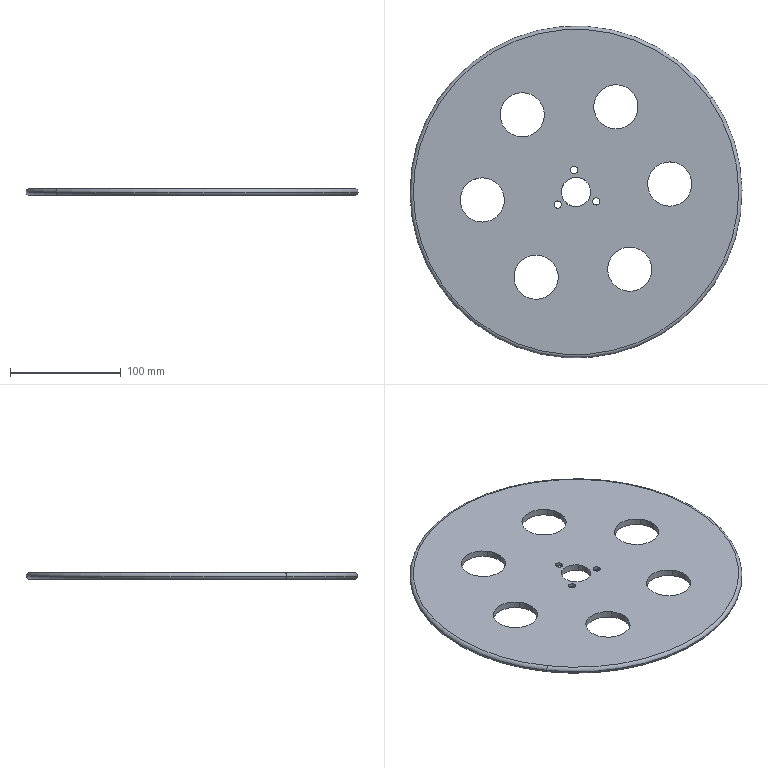Component | SolidWorks | JYTBJ-HeaderPlate-1 | 1 solid | 32 faces | box 300 x 300 x 6 mm | volume 370827 mm3 | cylinder 20 | cone 6 | torus 4 | plane 2 | commonest cylinder face diameters 40 x12 6.6 x6 26.5 x2
STEP:
#1=COLOUR_RGB('',0.7922,0.8196,0.9333);
#2=FILL_AREA_STYLE_COLOUR('',#1);
#3=FILL_AREA_STYLE('',(#2));
#4=SURFACE_STYLE_FILL_AREA(#3);
#5=SURFACE_SIDE_STYLE('',(#4));
#6=SURFACE_STYLE_USAGE(.BOTH.,#5);
#7=PRESENTATION_STYLE_ASSIGNMENT((#6));
#8=CARTESIAN_POINT('',(-2.556,3.98,1.909));
#9=VERTEX_POINT('',#8);
#10=CARTESIAN_POINT('',(-3.848,3.08,1.909));
#11=VERTEX_POINT('',#10);
#12=CARTESIAN_POINT('',(-3.202,3.53,1.909));
#13=DIRECTION('',(0.,0.,-1.));
#14=DIRECTION('',(0.08494,-0.9964,0.));
#15=AXIS2_PLACEMENT_3D('',#12,#13,#14);
#16=CIRCLE('',#15,0.7874);
#17=EDGE_CURVE('',#9,#11,#16,.T.);
#18=ORIENTED_EDGE('',*,*,#17,.F.);
#19=CARTESIAN_POINT('',(-2.556,3.98,1.673));
#20=VERTEX_POINT('',#19);
#21=CARTESIAN_POINT('',(-2.556,3.98,1.909));
#22=DIRECTION('',(0.,0.,-1.));
#23=VECTOR('',#22,39.37);
#24=LINE('',#21,#23);
#25=EDGE_CURVE('',#9,#20,#24,.T.);
#26=ORIENTED_EDGE('',*,*,#25,.T.);
#27=CARTESIAN_POINT('',(-3.848,3.08,1.673));
#28=VERTEX_POINT('',#27);
#29=CARTESIAN_POINT('',(-3.202,3.53,1.673));
#30=DIRECTION('',(0.,0.,-1.));
#31=DIRECTION('',(0.08494,-0.9964,0.));
#32=AXIS2_PLACEMENT_3D('',#29,#30,#31);
#33=CIRCLE('',#32,0.7874);
#34=EDGE_CURVE('',#20,#28,#33,.T.);
#35=ORIENTED_EDGE('',*,*,#34,.T.);
#36=CARTESIAN_POINT('',(-3.848,3.08,1.909));
#37=DIRECTION('',(0.,0.,-1.));
#38=VECTOR('',#37,39.37);
#39=LINE('',#36,#38);
#40=EDGE_CURVE('',#11,#28,#39,.T.);
#41=ORIENTED_EDGE('',*,*,#40,.F.);
#42=EDGE_LOOP('',(#18,#26,#35,#41));
#43=FACE_OUTER_BOUND('',#42,.T.);
#44=CARTESIAN_POINT('',(-3.202,3.53,1.909));
#45=DIRECTION('',(0.,0.,-1.));
#46=DIRECTION('',(-0.8204,-0.5718,0.));
#47=AXIS2_PLACEMENT_3D('',#44,#45,#46);
#48=CYLINDRICAL_SURFACE('',#47,0.7874);
#49=ADVANCED_FACE('',(#43),#48,.F.);
#50=CARTESIAN_POINT('',(-0.6422,1.235,1.909));
#51=VERTEX_POINT('',#50);
#52=CARTESIAN_POINT('',(-1.934,0.3341,1.909));
#53=VERTEX_POINT('',#52);
#54=CARTESIAN_POINT('',(-1.288,0.7843,1.909));
#55=DIRECTION('',(0.,0.,-1.));
#56=DIRECTION('',(0.9054,-0.4246,0.));
#57=AXIS2_PLACEMENT_3D('',#54,#55,#56);
#58=CIRCLE('',#57,0.7874);
#59=EDGE_CURVE('',#51,#53,#58,.T.);
#60=ORIENTED_EDGE('',*,*,#59,.F.);
#61=CARTESIAN_POINT('',(-0.6422,1.235,1.673));
#62=VERTEX_POINT('',#61);
#63=CARTESIAN_POINT('',(-0.6422,1.235,1.909));
#64=DIRECTION('',(0.,0.,-1.));
#65=VECTOR('',#64,39.37);
#66=LINE('',#63,#65);
#67=EDGE_CURVE('',#51,#62,#66,.T.);
#68=ORIENTED_EDGE('',*,*,#67,.T.);
#69=CARTESIAN_POINT('',(-1.934,0.3341,1.673));
#70=VERTEX_POINT('',#69);
#71=CARTESIAN_POINT('',(-1.288,0.7843,1.673));
#72=DIRECTION('',(0.,0.,-1.));
#73=DIRECTION('',(0.9054,-0.4246,0.));
#74=AXIS2_PLACEMENT_3D('',#71,#72,#73);
#75=CIRCLE('',#74,0.7874);
#76=EDGE_CURVE('',#62,#70,#75,.T.);
#77=ORIENTED_EDGE('',*,*,#76,.T.);
#78=CARTESIAN_POINT('',(-1.934,0.3341,1.909));
#79=DIRECTION('',(0.,0.,-1.));
#80=VECTOR('',#79,39.37);
#81=LINE('',#78,#80);
#82=EDGE_CURVE('',#53,#70,#81,.T.);
#83=ORIENTED_EDGE('',*,*,#82,.F.);
#84=EDGE_LOOP('',(#60,#68,#77,#83));
#85=FACE_OUTER_BOUND('',#84,.T.);
#86=CARTESIAN_POINT('',(-1.288,0.7843,1.909));
#87=DIRECTION('',(0.,0.,-1.));
#88=DIRECTION('',(-0.8204,-0.5718,0.));
#89=AXIS2_PLACEMENT_3D('',#86,#87,#88);
#90=CYLINDRICAL_SURFACE('',#89,0.7874);
#91=ADVANCED_FACE('',(#85),#90,.F.);
#92=CARTESIAN_POINT('',(2.692,1.519,1.909));
#93=VERTEX_POINT('',#92);
#94=CARTESIAN_POINT('',(1.4,0.6184,1.909));
#95=VERTEX_POINT('',#94);
#96=CARTESIAN_POINT('',(2.046,1.069,1.909));
#97=DIRECTION('',(0.,0.,-1.));
#98=DIRECTION('',(0.8204,0.5718,0.));
#99=AXIS2_PLACEMENT_3D('',#96,#97,#98);
#100=CIRCLE('',#99,0.7874);
#101=EDGE_CURVE('',#93,#95,#100,.T.);
#102=ORIENTED_EDGE('',*,*,#101,.F.);
#103=CARTESIAN_POINT('',(2.692,1.519,1.673));
#104=VERTEX_POINT('',#103);
#105=CARTESIAN_POINT('',(2.692,1.519,1.909));
#106=DIRECTION('',(0.,0.,-1.));
#107=VECTOR('',#106,39.37);
#108=LINE('',#105,#107);
#109=EDGE_CURVE('',#93,#104,#108,.T.);
#110=ORIENTED_EDGE('',*,*,#109,.T.);
#111=CARTESIAN_POINT('',(1.4,0.6184,1.673));
#112=VERTEX_POINT('',#111);
#113=CARTESIAN_POINT('',(2.046,1.069,1.673));
#114=DIRECTION('',(0.,0.,-1.));
#115=DIRECTION('',(0.8204,0.5718,0.));
#116=AXIS2_PLACEMENT_3D('',#113,#114,#115);
#117=CIRCLE('',#116,0.7874);
#118=EDGE_CURVE('',#104,#112,#117,.T.);
#119=ORIENTED_EDGE('',*,*,#118,.T.);
#120=CARTESIAN_POINT('',(1.4,0.6184,1.909));
#121=DIRECTION('',(0.,0.,-1.));
#122=VECTOR('',#121,39.37);
#123=LINE('',#120,#122);
#124=EDGE_CURVE('',#95,#112,#123,.T.);
#125=ORIENTED_EDGE('',*,*,#124,.F.);
#126=EDGE_LOOP('',(#102,#110,#119,#125));
#127=FACE_OUTER_BOUND('',#126,.T.);
#128=CARTESIAN_POINT('',(2.046,1.069,1.909));
#129=DIRECTION('',(0.,0.,-1.));
#130=DIRECTION('',(-0.8204,-0.5718,0.));
#131=AXIS2_PLACEMENT_3D('',#128,#129,#130);
#132=CYLINDRICAL_SURFACE('',#131,0.7874);
#133=ADVANCED_FACE('',(#127),#132,.F.);
#134=CARTESIAN_POINT('',(4.113,4.549,1.909));
#135=VERTEX_POINT('',#134);
#136=CARTESIAN_POINT('',(2.821,3.648,1.909));
#137=VERTEX_POINT('',#136);
#138=CARTESIAN_POINT('',(3.467,4.098,1.909));
#139=DIRECTION('',(0.,0.,-1.));
#140=DIRECTION('',(-0.08494,0.9964,0.));
#141=AXIS2_PLACEMENT_3D('',#138,#139,#140);
#142=CIRCLE('',#141,0.7874);
#143=EDGE_CURVE('',#135,#137,#142,.T.);
#144=ORIENTED_EDGE('',*,*,#143,.F.);
#145=CARTESIAN_POINT('',(4.113,4.549,1.673));
#146=VERTEX_POINT('',#145);
#147=CARTESIAN_POINT('',(4.113,4.549,1.909));
#148=DIRECTION('',(0.,0.,-1.));
#149=VECTOR('',#148,39.37);
#150=LINE('',#147,#149);
#151=EDGE_CURVE('',#135,#146,#150,.T.);
#152=ORIENTED_EDGE('',*,*,#151,.T.);
#153=CARTESIAN_POINT('',(2.821,3.648,1.673));
#154=VERTEX_POINT('',#153);
#155=CARTESIAN_POINT('',(3.467,4.098,1.673));
#156=DIRECTION('',(0.,0.,-1.));
#157=DIRECTION('',(-0.08494,0.9964,0.));
#158=AXIS2_PLACEMENT_3D('',#155,#156,#157);
#159=CIRCLE('',#158,0.7874);
#160=EDGE_CURVE('',#146,#154,#159,.T.);
#161=ORIENTED_EDGE('',*,*,#160,.T.);
#162=CARTESIAN_POINT('',(2.821,3.648,1.909));
#163=DIRECTION('',(0.,0.,-1.));
#164=VECTOR('',#163,39.37);
#165=LINE('',#162,#164);
#166=EDGE_CURVE('',#137,#154,#165,.T.);
#167=ORIENTED_EDGE('',*,*,#166,.F.);
#168=EDGE_LOOP('',(#144,#152,#161,#167));
#169=FACE_OUTER_BOUND('',#168,.T.);
#170=CARTESIAN_POINT('',(3.467,4.098,1.909));
#171=DIRECTION('',(0.,0.,-1.));
#172=DIRECTION('',(-0.8204,-0.5718,0.));
#173=AXIS2_PLACEMENT_3D('',#170,#171,#172);
#174=CYLINDRICAL_SURFACE('',#173,0.7874);
#175=ADVANCED_FACE('',(#169),#174,.F.);
#176=CARTESIAN_POINT('',(2.2,7.294,1.909));
#177=VERTEX_POINT('',#176);
#178=CARTESIAN_POINT('',(0.9078,6.394,1.909));
#179=VERTEX_POINT('',#178);
#180=CARTESIAN_POINT('',(1.554,6.844,1.909));
#181=DIRECTION('',(0.,0.,-1.));
#182=DIRECTION('',(-0.9054,0.4246,0.));
#183=AXIS2_PLACEMENT_3D('',#180,#181,#182);
#184=CIRCLE('',#183,0.7874);
#185=EDGE_CURVE('',#177,#179,#184,.T.);
#186=ORIENTED_EDGE('',*,*,#185,.F.);
#187=CARTESIAN_POINT('',(2.2,7.294,1.673));
#188=VERTEX_POINT('',#187);
#189=CARTESIAN_POINT('',(2.2,7.294,1.909));
#190=DIRECTION('',(0.,0.,-1.));
#191=VECTOR('',#190,39.37);
#192=LINE('',#189,#191);
#193=EDGE_CURVE('',#177,#188,#192,.T.);
#194=ORIENTED_EDGE('',*,*,#193,.T.);
#195=CARTESIAN_POINT('',(0.9078,6.394,1.673));
#196=VERTEX_POINT('',#195);
#197=CARTESIAN_POINT('',(1.554,6.844,1.673));
#198=DIRECTION('',(0.,0.,-1.));
#199=DIRECTION('',(-0.9054,0.4246,0.));
#200=AXIS2_PLACEMENT_3D('',#197,#198,#199);
#201=CIRCLE('',#200,0.7874);
#202=EDGE_CURVE('',#188,#196,#201,.T.);
#203=ORIENTED_EDGE('',*,*,#202,.T.);
#204=CARTESIAN_POINT('',(0.9078,6.394,1.909));
#205=DIRECTION('',(0.,0.,-1.));
#206=VECTOR('',#205,39.37);
#207=LINE('',#204,#206);
#208=EDGE_CURVE('',#179,#196,#207,.T.);
#209=ORIENTED_EDGE('',*,*,#208,.F.);
#210=EDGE_LOOP('',(#186,#194,#203,#209));
#211=FACE_OUTER_BOUND('',#210,.T.);
#212=CARTESIAN_POINT('',(1.554,6.844,1.909));
#213=DIRECTION('',(0.,0.,-1.));
#214=DIRECTION('',(-0.8204,-0.5718,0.));
#215=AXIS2_PLACEMENT_3D('',#212,#213,#214);
#216=CYLINDRICAL_SURFACE('',#215,0.7874);
#217=ADVANCED_FACE('',(#211),#216,.F.);
#218=CARTESIAN_POINT('',(4.881,7.123,1.909));
#219=VERTEX_POINT('',#218);
#220=CARTESIAN_POINT('',(-4.615,0.5051,1.909));
#221=VERTEX_POINT('',#220);
#222=CARTESIAN_POINT('',(0.1328,3.814,1.909));
#223=DIRECTION('',(-0.,-0.,1.));
#224=DIRECTION('',(-0.8204,-0.5718,0.));
#225=AXIS2_PLACEMENT_3D('',#222,#223,#224);
#226=CIRCLE('',#225,5.787);
#227=EDGE_CURVE('',#219,#221,#226,.T.);
#228=ORIENTED_EDGE('',*,*,#227,.F.);
#229=CARTESIAN_POINT('',(4.978,7.191,1.791));
#230=VERTEX_POINT('',#229);
#231=CARTESIAN_POINT('',(4.881,7.123,1.791));
#232=DIRECTION('',(-0.5718,0.8204,0.));
#233=DIRECTION('',(-0.8204,-0.5718,0.));
#234=AXIS2_PLACEMENT_3D('',#231,#232,#233);
#235=CIRCLE('',#234,0.1181);
#236=EDGE_CURVE('',#219,#230,#235,.T.);
#237=ORIENTED_EDGE('',*,*,#236,.T.);
#238=CARTESIAN_POINT('',(-4.712,0.4376,1.791));
#239=VERTEX_POINT('',#238);
#240=CARTESIAN_POINT('',(0.1328,3.814,1.791));
#241=DIRECTION('',(-0.,-0.,1.));
#242=DIRECTION('',(-0.8204,-0.5718,0.));
#243=AXIS2_PLACEMENT_3D('',#240,#241,#242);
#244=CIRCLE('',#243,5.906);
#245=EDGE_CURVE('',#230,#239,#244,.T.);
#246=ORIENTED_EDGE('',*,*,#245,.T.);
#247=CARTESIAN_POINT('',(-4.615,0.5051,1.791));
#248=DIRECTION('',(0.5718,-0.8204,-0.));
#249=DIRECTION('',(0.8204,0.5718,0.));
#250=AXIS2_PLACEMENT_3D('',#247,#248,#249);
#251=CIRCLE('',#250,0.1181);
#252=EDGE_CURVE('',#221,#239,#251,.T.);
#253=ORIENTED_EDGE('',*,*,#252,.F.);
#254=EDGE_LOOP('',(#228,#237,#246,#253));
#255=FACE_OUTER_BOUND('',#254,.T.);
#256=CARTESIAN_POINT('',(0.1328,3.814,1.791));
#257=DIRECTION('',(0.,0.,-1.));
#258=DIRECTION('',(-0.8204,-0.5718,-0.));
#259=AXIS2_PLACEMENT_3D('',#256,#257,#258);
#260=TOROIDAL_SURFACE('',#259,5.787,0.1181);
#261=ADVANCED_FACE('',(#255),#260,.T.);
#262=ORIENTED_EDGE('',*,*,#245,.F.);
#263=CARTESIAN_POINT('',(4.881,7.123,1.673));
#264=VERTEX_POINT('',#263);
#265=CARTESIAN_POINT('',(4.881,7.123,1.791));
#266=DIRECTION('',(-0.5718,0.8204,0.));
#267=DIRECTION('',(-0.8204,-0.5718,0.));
#268=AXIS2_PLACEMENT_3D('',#265,#266,#267);
#269=CIRCLE('',#268,0.1181);
#270=EDGE_CURVE('',#230,#264,#269,.T.);
#271=ORIENTED_EDGE('',*,*,#270,.T.);
#272=CARTESIAN_POINT('',(-4.615,0.5051,1.673));
#273=VERTEX_POINT('',#272);
#274=CARTESIAN_POINT('',(0.1328,3.814,1.673));
#275=DIRECTION('',(0.,0.,-1.));
#276=DIRECTION('',(-0.8204,-0.5718,0.));
#277=AXIS2_PLACEMENT_3D('',#274,#275,#276);
#278=CIRCLE('',#277,5.787);
#279=EDGE_CURVE('',#273,#264,#278,.T.);
#280=ORIENTED_EDGE('',*,*,#279,.F.);
#281=CARTESIAN_POINT('',(-4.615,0.5051,1.791));
#282=DIRECTION('',(0.5718,-0.8204,-0.));
#283=DIRECTION('',(0.8204,0.5718,0.));
#284=AXIS2_PLACEMENT_3D('',#281,#282,#283);
#285=CIRCLE('',#284,0.1181);
#286=EDGE_CURVE('',#239,#273,#285,.T.);
#287=ORIENTED_EDGE('',*,*,#286,.F.);
#288=EDGE_LOOP('',(#262,#271,#280,#287));
#289=FACE_OUTER_BOUND('',#288,.T.);
#290=CARTESIAN_POINT('',(0.1328,3.814,1.791));
#291=DIRECTION('',(0.,0.,-1.));
#292=DIRECTION('',(-0.8204,-0.5718,-0.));
#293=AXIS2_PLACEMENT_3D('',#290,#291,#292);
#294=TOROIDAL_SURFACE('',#293,5.787,0.1181);
#295=ADVANCED_FACE('',(#289),#294,.T.);
#296=CARTESIAN_POINT('',(-1.135,7.01,1.909));
#297=VERTEX_POINT('',#296);
#298=CARTESIAN_POINT('',(-2.427,6.109,1.909));
#299=VERTEX_POINT('',#298);
#300=CARTESIAN_POINT('',(-1.781,6.56,1.909));
#301=DIRECTION('',(0.,0.,-1.));
#302=DIRECTION('',(-0.8204,-0.5718,0.));
#303=AXIS2_PLACEMENT_3D('',#300,#301,#302);
#304=CIRCLE('',#303,0.7874);
#305=EDGE_CURVE('',#297,#299,#304,.T.);
#306=ORIENTED_EDGE('',*,*,#305,.F.);
#307=CARTESIAN_POINT('',(-1.135,7.01,1.673));
#308=VERTEX_POINT('',#307);
#309=CARTESIAN_POINT('',(-1.135,7.01,1.909));
#310=DIRECTION('',(0.,0.,-1.));
#311=VECTOR('',#310,39.37);
#312=LINE('',#309,#311);
#313=EDGE_CURVE('',#297,#308,#312,.T.);
#314=ORIENTED_EDGE('',*,*,#313,.T.);
#315=CARTESIAN_POINT('',(-2.427,6.109,1.673));
#316=VERTEX_POINT('',#315);
#317=CARTESIAN_POINT('',(-1.781,6.56,1.673));
#318=DIRECTION('',(0.,0.,-1.));
#319=DIRECTION('',(-0.8204,-0.5718,0.));
#320=AXIS2_PLACEMENT_3D('',#317,#318,#319);
#321=CIRCLE('',#320,0.7874);
#322=EDGE_CURVE('',#308,#316,#321,.T.);
#323=ORIENTED_EDGE('',*,*,#322,.T.);
#324=CARTESIAN_POINT('',(-2.427,6.109,1.909));
#325=DIRECTION('',(0.,0.,-1.));
#326=VECTOR('',#325,39.37);
#327=LINE('',#324,#326);
#328=EDGE_CURVE('',#299,#316,#327,.T.);
#329=ORIENTED_EDGE('',*,*,#328,.F.);
#330=EDGE_LOOP('',(#306,#314,#323,#329));
#331=FACE_OUTER_BOUND('',#330,.T.);
#332=CARTESIAN_POINT('',(-1.781,6.56,1.909));
#333=DIRECTION('',(0.,0.,-1.));
#334=DIRECTION('',(-0.8204,-0.5718,0.));
#335=AXIS2_PLACEMENT_3D('',#332,#333,#334);
#336=CYLINDRICAL_SURFACE('',#335,0.7874);
#337=ADVANCED_FACE('',(#331),#336,.F.);
#338=CARTESIAN_POINT('',(0.9523,3.554,1.809));
#339=VERTEX_POINT('',#338);
#340=CARTESIAN_POINT('',(0.7391,3.405,1.809));
#341=VERTEX_POINT('',#340);
#342=CARTESIAN_POINT('',(0.8457,3.48,1.809));
#343=DIRECTION('',(0.,0.,-1.));
#344=DIRECTION('',(-0.8204,-0.5718,0.));
#345=AXIS2_PLACEMENT_3D('',#342,#343,#344);
#346=CIRCLE('',#345,0.1299);
#347=EDGE_CURVE('',#339,#341,#346,.T.);
#348=ORIENTED_EDGE('',*,*,#347,.F.);
#349=CARTESIAN_POINT('',(1.064,3.632,1.673));
#350=VERTEX_POINT('',#349);
#351=CARTESIAN_POINT('',(1.064,3.632,1.673));
#352=DIRECTION('',(0.5801,0.4043,-0.7071));
#353=VECTOR('',#352,39.37);
#354=LINE('',#351,#353);
#355=EDGE_CURVE('',#339,#350,#354,.T.);
#356=ORIENTED_EDGE('',*,*,#355,.T.);
#357=CARTESIAN_POINT('',(0.6277,3.328,1.673));
#358=VERTEX_POINT('',#357);
#359=CARTESIAN_POINT('',(0.8457,3.48,1.673));
#360=DIRECTION('',(0.,0.,-1.));
#361=DIRECTION('',(-0.8204,-0.5718,0.));
#362=AXIS2_PLACEMENT_3D('',#359,#360,#361);
#363=CIRCLE('',#362,0.2657);
#364=EDGE_CURVE('',#350,#358,#363,.T.);
#365=ORIENTED_EDGE('',*,*,#364,.T.);
#366=CARTESIAN_POINT('',(0.6277,3.328,1.673));
#367=DIRECTION('',(-0.5801,-0.4043,-0.7071));
#368=VECTOR('',#367,39.37);
#369=LINE('',#366,#368);
#370=EDGE_CURVE('',#341,#358,#369,.T.);
#371=ORIENTED_EDGE('',*,*,#370,.F.);
#372=EDGE_LOOP('',(#348,#356,#365,#371));
#373=FACE_OUTER_BOUND('',#372,.T.);
#374=CARTESIAN_POINT('',(0.8457,3.48,1.673));
#375=DIRECTION('',(0.,0.,-1.));
#376=DIRECTION('',(-0.8204,-0.5718,0.));
#377=AXIS2_PLACEMENT_3D('',#374,#375,#376);
#378=CONICAL_SURFACE('',#377,0.2657,0.7854);
#379=ADVANCED_FACE('',(#373),#378,.F.);
#380=CARTESIAN_POINT('',(0.9523,3.554,1.909));
#381=VERTEX_POINT('',#380);
#382=CARTESIAN_POINT('',(0.7391,3.405,1.909));
#383=VERTEX_POINT('',#382);
#384=CARTESIAN_POINT('',(0.8457,3.48,1.909));
#385=DIRECTION('',(0.,0.,-1.));
#386=DIRECTION('',(-0.8204,-0.5718,0.));
#387=AXIS2_PLACEMENT_3D('',#384,#385,#386);
#388=CIRCLE('',#387,0.1299);
#389=EDGE_CURVE('',#381,#383,#388,.T.);
#390=ORIENTED_EDGE('',*,*,#389,.F.);
#391=CARTESIAN_POINT('',(0.9523,3.554,1.673));
#392=DIRECTION('',(0.,0.,-1.));
#393=VECTOR('',#392,39.37);
#394=LINE('',#391,#393);
#395=EDGE_CURVE('',#381,#339,#394,.T.);
#396=ORIENTED_EDGE('',*,*,#395,.T.);
#397=ORIENTED_EDGE('',*,*,#347,.T.);
#398=CARTESIAN_POINT('',(0.7391,3.405,1.673));
#399=DIRECTION('',(0.,0.,-1.));
#400=VECTOR('',#399,39.37);
#401=LINE('',#398,#400);
#402=EDGE_CURVE('',#383,#341,#401,.T.);
#403=ORIENTED_EDGE('',*,*,#402,.F.);
#404=EDGE_LOOP('',(#390,#396,#397,#403));
#405=FACE_OUTER_BOUND('',#404,.T.);
#406=CARTESIAN_POINT('',(0.8457,3.48,1.673));
#407=DIRECTION('',(0.,0.,-1.));
#408=DIRECTION('',(-0.8204,-0.5718,0.));
#409=AXIS2_PLACEMENT_3D('',#406,#407,#408);
#410=CYLINDRICAL_SURFACE('',#409,0.1299);
#411=ADVANCED_FACE('',(#405),#410,.F.);
#412=CARTESIAN_POINT('',(0.1725,4.673,1.809));
#413=VERTEX_POINT('',#412);
#414=CARTESIAN_POINT('',(-0.04066,4.524,1.809));
#415=VERTEX_POINT('',#414);
#416=CARTESIAN_POINT('',(0.06593,4.599,1.809));
#417=DIRECTION('',(0.,0.,-1.));
#418=DIRECTION('',(-0.8204,-0.5718,0.));
#419=AXIS2_PLACEMENT_3D('',#416,#417,#418);
#420=CIRCLE('',#419,0.1299);
#421=EDGE_CURVE('',#413,#415,#420,.T.);
#422=ORIENTED_EDGE('',*,*,#421,.F.);
#423=CARTESIAN_POINT('',(0.284,4.751,1.673));
#424=VERTEX_POINT('',#423);
#425=CARTESIAN_POINT('',(0.284,4.751,1.673));
#426=DIRECTION('',(0.5801,0.4043,-0.7071));
#427=VECTOR('',#426,39.37);
#428=LINE('',#425,#427);
#429=EDGE_CURVE('',#413,#424,#428,.T.);
#430=ORIENTED_EDGE('',*,*,#429,.T.);
#431=CARTESIAN_POINT('',(0.0885,4.334,1.673));
#432=VERTEX_POINT('',#431);
#433=CARTESIAN_POINT('',(0.06593,4.599,1.673));
#434=DIRECTION('',(0.,0.,-1.));
#435=DIRECTION('',(-0.8204,-0.5718,0.));
#436=AXIS2_PLACEMENT_3D('',#433,#434,#435);
#437=CIRCLE('',#436,0.2657);
#438=EDGE_CURVE('',#424,#432,#437,.T.);
#439=ORIENTED_EDGE('',*,*,#438,.T.);
#440=CARTESIAN_POINT('',(-0.1521,4.447,1.673));
#441=VERTEX_POINT('',#440);
#442=CARTESIAN_POINT('',(0.06593,4.599,1.673));
#443=DIRECTION('',(0.,0.,-1.));
#444=DIRECTION('',(-0.8204,-0.5718,0.));
#445=AXIS2_PLACEMENT_3D('',#442,#443,#444);
#446=CIRCLE('',#445,0.2657);
#447=EDGE_CURVE('',#432,#441,#446,.T.);
#448=ORIENTED_EDGE('',*,*,#447,.T.);
#449=CARTESIAN_POINT('',(-0.1521,4.447,1.673));
#450=DIRECTION('',(-0.5801,-0.4043,-0.7071));
#451=VECTOR('',#450,39.37);
#452=LINE('',#449,#451);
#453=EDGE_CURVE('',#415,#441,#452,.T.);
#454=ORIENTED_EDGE('',*,*,#453,.F.);
#455=EDGE_LOOP('',(#422,#430,#439,#448,#454));
#456=FACE_OUTER_BOUND('',#455,.T.);
#457=CARTESIAN_POINT('',(0.06593,4.599,1.673));
#458=DIRECTION('',(0.,0.,-1.));
#459=DIRECTION('',(-0.8204,-0.5718,0.));
#460=AXIS2_PLACEMENT_3D('',#457,#458,#459);
#461=CONICAL_SURFACE('',#460,0.2657,0.7854);
#462=ADVANCED_FACE('',(#456),#461,.F.);
#463=CARTESIAN_POINT('',(0.1725,4.673,1.909));
#464=VERTEX_POINT('',#463);
#465=CARTESIAN_POINT('',(-0.04066,4.524,1.909));
#466=VERTEX_POINT('',#465);
#467=CARTESIAN_POINT('',(0.06593,4.599,1.909));
#468=DIRECTION('',(0.,0.,-1.));
#469=DIRECTION('',(-0.8204,-0.5718,0.));
#470=AXIS2_PLACEMENT_3D('',#467,#468,#469);
#471=CIRCLE('',#470,0.1299);
#472=EDGE_CURVE('',#464,#466,#471,.T.);
#473=ORIENTED_EDGE('',*,*,#472,.F.);
#474=CARTESIAN_POINT('',(0.1725,4.673,1.673));
#475=DIRECTION('',(0.,0.,-1.));
#476=VECTOR('',#475,39.37);
#477=LINE('',#474,#476);
#478=EDGE_CURVE('',#464,#413,#477,.T.);
#479=ORIENTED_EDGE('',*,*,#478,.T.);
#480=ORIENTED_EDGE('',*,*,#421,.T.);
#481=CARTESIAN_POINT('',(-0.04066,4.524,1.673));
#482=DIRECTION('',(0.,0.,-1.));
#483=VECTOR('',#482,39.37);
#484=LINE('',#481,#483);
#485=EDGE_CURVE('',#466,#415,#484,.T.);
#486=ORIENTED_EDGE('',*,*,#485,.F.);
#487=EDGE_LOOP('',(#473,#479,#480,#486));
#488=FACE_OUTER_BOUND('',#487,.T.);
#489=CARTESIAN_POINT('',(0.06593,4.599,1.673));
#490=DIRECTION('',(0.,0.,-1.));
#491=DIRECTION('',(-0.8204,-0.5718,0.));
#492=AXIS2_PLACEMENT_3D('',#489,#490,#491);
#493=CYLINDRICAL_SURFACE('',#492,0.1299);
#494=ADVANCED_FACE('',(#488),#493,.F.);
#495=CARTESIAN_POINT('',(-0.4066,3.438,1.809));
#496=VERTEX_POINT('',#495);
#497=CARTESIAN_POINT('',(-0.6198,3.29,1.809));
#498=VERTEX_POINT('',#497);
#499=CARTESIAN_POINT('',(-0.5132,3.364,1.809));
#500=DIRECTION('',(0.,0.,-1.));
#501=DIRECTION('',(-0.8204,-0.5718,0.));
#502=AXIS2_PLACEMENT_3D('',#499,#500,#501);
#503=CIRCLE('',#502,0.1299);
#504=EDGE_CURVE('',#496,#498,#503,.T.);
#505=ORIENTED_EDGE('',*,*,#504,.F.);
#506=CARTESIAN_POINT('',(-0.2952,3.516,1.673));
#507=VERTEX_POINT('',#506);
#508=CARTESIAN_POINT('',(-0.2952,3.516,1.673));
#509=DIRECTION('',(0.5801,0.4043,-0.7071));
#510=VECTOR('',#509,39.37);
#511=LINE('',#508,#510);
#512=EDGE_CURVE('',#496,#507,#511,.T.);
#513=ORIENTED_EDGE('',*,*,#512,.T.);
#514=CARTESIAN_POINT('',(-0.7312,3.212,1.673));
#515=VERTEX_POINT('',#514);
#516=CARTESIAN_POINT('',(-0.5132,3.364,1.673));
#517=DIRECTION('',(0.,0.,-1.));
#518=DIRECTION('',(-0.8204,-0.5718,0.));
#519=AXIS2_PLACEMENT_3D('',#516,#517,#518);
#520=CIRCLE('',#519,0.2657);
#521=EDGE_CURVE('',#507,#515,#520,.T.);
#522=ORIENTED_EDGE('',*,*,#521,.T.);
#523=CARTESIAN_POINT('',(-0.7312,3.212,1.673));
#524=DIRECTION('',(-0.5801,-0.4043,-0.7071));
#525=VECTOR('',#524,39.37);
#526=LINE('',#523,#525);
#527=EDGE_CURVE('',#498,#515,#526,.T.);
#528=ORIENTED_EDGE('',*,*,#527,.F.);
#529=EDGE_LOOP('',(#505,#513,#522,#528));
#530=FACE_OUTER_BOUND('',#529,.T.);
#531=CARTESIAN_POINT('',(-0.5132,3.364,1.673));
#532=DIRECTION('',(0.,0.,-1.));
#533=DIRECTION('',(-0.8204,-0.5718,0.));
#534=AXIS2_PLACEMENT_3D('',#531,#532,#533);
#535=CONICAL_SURFACE('',#534,0.2657,0.7854);
#536=ADVANCED_FACE('',(#530),#535,.F.);
#537=CARTESIAN_POINT('',(-0.4066,3.438,1.909));
#538=VERTEX_POINT('',#537);
#539=CARTESIAN_POINT('',(-0.6198,3.29,1.909));
#540=VERTEX_POINT('',#539);
#541=CARTESIAN_POINT('',(-0.5132,3.364,1.909));
#542=DIRECTION('',(0.,0.,-1.));
#543=DIRECTION('',(-0.8204,-0.5718,0.));
#544=AXIS2_PLACEMENT_3D('',#541,#542,#543);
#545=CIRCLE('',#544,0.1299);
#546=EDGE_CURVE('',#538,#540,#545,.T.);
#547=ORIENTED_EDGE('',*,*,#546,.F.);
#548=CARTESIAN_POINT('',(-0.4066,3.438,1.673));
#549=DIRECTION('',(0.,0.,-1.));
#550=VECTOR('',#549,39.37);
#551=LINE('',#548,#550);
#552=EDGE_CURVE('',#538,#496,#551,.T.);
#553=ORIENTED_EDGE('',*,*,#552,.T.);
#554=ORIENTED_EDGE('',*,*,#504,.T.);
#555=CARTESIAN_POINT('',(-0.6198,3.29,1.673));
#556=DIRECTION('',(0.,0.,-1.));
#557=VECTOR('',#556,39.37);
#558=LINE('',#555,#557);
#559=EDGE_CURVE('',#540,#498,#558,.T.);
#560=ORIENTED_EDGE('',*,*,#559,.F.);
#561=EDGE_LOOP('',(#547,#553,#554,#560));
#562=FACE_OUTER_BOUND('',#561,.T.);
#563=CARTESIAN_POINT('',(-0.5132,3.364,1.673));
#564=DIRECTION('',(0.,0.,-1.));
#565=DIRECTION('',(-0.8204,-0.5718,0.));
#566=AXIS2_PLACEMENT_3D('',#563,#564,#565);
#567=CYLINDRICAL_SURFACE('',#566,0.1299);
#568=ADVANCED_FACE('',(#562),#567,.F.);
#569=CARTESIAN_POINT('',(0.5608,4.112,1.909));
#570=VERTEX_POINT('',#569);
#571=CARTESIAN_POINT('',(-0.2952,3.516,1.909));
#572=VERTEX_POINT('',#571);
#573=CARTESIAN_POINT('',(0.1328,3.814,1.909));
#574=DIRECTION('',(0.,0.,-1.));
#575=DIRECTION('',(-0.8204,-0.5718,0.));
#576=AXIS2_PLACEMENT_3D('',#573,#574,#575);
#577=CIRCLE('',#576,0.5217);
#578=EDGE_CURVE('',#570,#572,#577,.T.);
#579=ORIENTED_EDGE('',*,*,#578,.F.);
#580=CARTESIAN_POINT('',(0.5608,4.112,1.673));
#581=VERTEX_POINT('',#580);
#582=CARTESIAN_POINT('',(0.5608,4.112,1.909));
#583=DIRECTION('',(0.,0.,-1.));
#584=VECTOR('',#583,39.37);
#585=LINE('',#582,#584);
#586=EDGE_CURVE('',#570,#581,#585,.T.);
#587=ORIENTED_EDGE('',*,*,#586,.T.);
#588=CARTESIAN_POINT('',(0.6051,3.593,1.673));
#589=VERTEX_POINT('',#588);
#590=CARTESIAN_POINT('',(0.1328,3.814,1.673));
#591=DIRECTION('',(0.,0.,-1.));
#592=DIRECTION('',(-0.8204,-0.5718,0.));
#593=AXIS2_PLACEMENT_3D('',#590,#591,#592);
#594=CIRCLE('',#593,0.5217);
#595=EDGE_CURVE('',#581,#589,#594,.T.);
#596=ORIENTED_EDGE('',*,*,#595,.T.);
#597=CARTESIAN_POINT('',(0.1328,3.814,1.673));
#598=DIRECTION('',(0.,0.,-1.));
#599=DIRECTION('',(-0.8204,-0.5718,0.));
#600=AXIS2_PLACEMENT_3D('',#597,#598,#599);
#601=CIRCLE('',#600,0.5217);
#602=EDGE_CURVE('',#589,#507,#601,.T.);
#603=ORIENTED_EDGE('',*,*,#602,.T.);
#604=CARTESIAN_POINT('',(-0.2952,3.516,1.909));
#605=DIRECTION('',(0.,0.,-1.));
#606=VECTOR('',#605,39.37);
#607=LINE('',#604,#606);
#608=EDGE_CURVE('',#572,#507,#607,.T.);
#609=ORIENTED_EDGE('',*,*,#608,.F.);
#610=EDGE_LOOP('',(#579,#587,#596,#603,#609));
#611=FACE_OUTER_BOUND('',#610,.T.);
#612=CARTESIAN_POINT('',(0.1328,3.814,1.909));
#613=DIRECTION('',(0.,0.,-1.));
#614=DIRECTION('',(-0.8204,-0.5718,0.));
#615=AXIS2_PLACEMENT_3D('',#612,#613,#614);
#616=CYLINDRICAL_SURFACE('',#615,0.5217);
#617=ADVANCED_FACE('',(#611),#616,.F.);
#618=CARTESIAN_POINT('',(-3.202,3.53,1.673));
#619=DIRECTION('',(0.,0.,-1.));
#620=DIRECTION('',(0.08494,-0.9964,0.));
#621=AXIS2_PLACEMENT_3D('',#618,#619,#620);
#622=CIRCLE('',#621,0.7874);
#623=EDGE_CURVE('',#28,#20,#622,.T.);
#624=ORIENTED_EDGE('',*,*,#623,.F.);
#625=ORIENTED_EDGE('',*,*,#34,.F.);
#626=EDGE_LOOP('',(#624,#625));
#627=FACE_BOUND('',#626,.T.);
#628=CARTESIAN_POINT('',(-1.288,0.7843,1.673));
#629=DIRECTION('',(0.,0.,-1.));
#630=DIRECTION('',(0.9054,-0.4246,0.));
#631=AXIS2_PLACEMENT_3D('',#628,#629,#630);
#632=CIRCLE('',#631,0.7874);
#633=EDGE_CURVE('',#70,#62,#632,.T.);
#634=ORIENTED_EDGE('',*,*,#633,.F.);
#635=ORIENTED_EDGE('',*,*,#76,.F.);
#636=EDGE_LOOP('',(#634,#635));
#637=FACE_BOUND('',#636,.T.);
#638=CARTESIAN_POINT('',(2.046,1.069,1.673));
#639=DIRECTION('',(0.,0.,-1.));
#640=DIRECTION('',(0.8204,0.5718,0.));
#641=AXIS2_PLACEMENT_3D('',#638,#639,#640);
#642=CIRCLE('',#641,0.7874);
#643=EDGE_CURVE('',#112,#104,#642,.T.);
#644=ORIENTED_EDGE('',*,*,#643,.F.);
#645=ORIENTED_EDGE('',*,*,#118,.F.);
#646=EDGE_LOOP('',(#644,#645));
#647=FACE_BOUND('',#646,.T.);
#648=CARTESIAN_POINT('',(3.467,4.098,1.673));
#649=DIRECTION('',(0.,0.,-1.));
#650=DIRECTION('',(-0.08494,0.9964,0.));
#651=AXIS2_PLACEMENT_3D('',#648,#649,#650);
#652=CIRCLE('',#651,0.7874);
#653=EDGE_CURVE('',#154,#146,#652,.T.);
#654=ORIENTED_EDGE('',*,*,#653,.F.);
#655=ORIENTED_EDGE('',*,*,#160,.F.);
#656=EDGE_LOOP('',(#654,#655));
#657=FACE_BOUND('',#656,.T.);
#658=CARTESIAN_POINT('',(1.554,6.844,1.673));
#659=DIRECTION('',(0.,0.,-1.));
#660=DIRECTION('',(-0.9054,0.4246,0.));
#661=AXIS2_PLACEMENT_3D('',#658,#659,#660);
#662=CIRCLE('',#661,0.7874);
#663=EDGE_CURVE('',#196,#188,#662,.T.);
#664=ORIENTED_EDGE('',*,*,#663,.F.);
#665=ORIENTED_EDGE('',*,*,#202,.F.);
#666=EDGE_LOOP('',(#664,#665));
#667=FACE_BOUND('',#666,.T.);
#668=ORIENTED_EDGE('',*,*,#279,.T.);
#669=CARTESIAN_POINT('',(0.1328,3.814,1.673));
#670=DIRECTION('',(0.,0.,-1.));
#671=DIRECTION('',(-0.8204,-0.5718,0.));
#672=AXIS2_PLACEMENT_3D('',#669,#670,#671);
#673=CIRCLE('',#672,5.787);
#674=EDGE_CURVE('',#264,#273,#673,.T.);
#675=ORIENTED_EDGE('',*,*,#674,.T.);
#676=EDGE_LOOP('',(#668,#675));
#677=FACE_OUTER_BOUND('',#676,.T.);
#678=CARTESIAN_POINT('',(-1.781,6.56,1.673));
#679=DIRECTION('',(0.,0.,-1.));
#680=DIRECTION('',(-0.8204,-0.5718,0.));
#681=AXIS2_PLACEMENT_3D('',#678,#679,#680);
#682=CIRCLE('',#681,0.7874);
#683=EDGE_CURVE('',#316,#308,#682,.T.);
#684=ORIENTED_EDGE('',*,*,#683,.F.);
#685=ORIENTED_EDGE('',*,*,#322,.F.);
#686=EDGE_LOOP('',(#684,#685));
#687=FACE_BOUND('',#686,.T.);
#688=ORIENTED_EDGE('',*,*,#602,.F.);
#689=CARTESIAN_POINT('',(0.8457,3.48,1.673));
#690=DIRECTION('',(0.,0.,-1.));
#691=DIRECTION('',(-0.8204,-0.5718,0.));
#692=AXIS2_PLACEMENT_3D('',#689,#690,#691);
#693=CIRCLE('',#692,0.2657);
#694=EDGE_CURVE('',#358,#589,#693,.T.);
#695=ORIENTED_EDGE('',*,*,#694,.F.);
#696=ORIENTED_EDGE('',*,*,#364,.F.);
#697=CARTESIAN_POINT('',(0.8457,3.48,1.673));
#698=DIRECTION('',(0.,0.,-1.));
#699=DIRECTION('',(-0.8204,-0.5718,0.));
#700=AXIS2_PLACEMENT_3D('',#697,#698,#699);
#701=CIRCLE('',#700,0.2657);
#702=EDGE_CURVE('',#589,#350,#701,.T.);
#703=ORIENTED_EDGE('',*,*,#702,.F.);
#704=ORIENTED_EDGE('',*,*,#595,.F.);
#705=CARTESIAN_POINT('',(0.1328,3.814,1.673));
#706=DIRECTION('',(0.,0.,-1.));
#707=DIRECTION('',(-0.8204,-0.5718,0.));
#708=AXIS2_PLACEMENT_3D('',#705,#706,#707);
#709=CIRCLE('',#708,0.5217);
#710=EDGE_CURVE('',#432,#581,#709,.T.);
#711=ORIENTED_EDGE('',*,*,#710,.F.);
#712=ORIENTED_EDGE('',*,*,#438,.F.);
#713=CARTESIAN_POINT('',(0.06593,4.599,1.673));
#714=DIRECTION('',(0.,0.,-1.));
#715=DIRECTION('',(-0.8204,-0.5718,0.));
#716=AXIS2_PLACEMENT_3D('',#713,#714,#715);
#717=CIRCLE('',#716,0.2657);
#718=EDGE_CURVE('',#441,#424,#717,.T.);
#719=ORIENTED_EDGE('',*,*,#718,.F.);
#720=ORIENTED_EDGE('',*,*,#447,.F.);
#721=CARTESIAN_POINT('',(0.1328,3.814,1.673));
#722=DIRECTION('',(0.,0.,-1.));
#723=DIRECTION('',(-0.8204,-0.5718,0.));
#724=AXIS2_PLACEMENT_3D('',#721,#722,#723);
#725=CIRCLE('',#724,0.5217);
#726=EDGE_CURVE('',#507,#432,#725,.T.);
#727=ORIENTED_EDGE('',*,*,#726,.F.);
#728=CARTESIAN_POINT('',(-0.5132,3.364,1.673));
#729=DIRECTION('',(0.,0.,-1.));
#730=DIRECTION('',(-0.8204,-0.5718,0.));
#731=AXIS2_PLACEMENT_3D('',#728,#729,#730);
#732=CIRCLE('',#731,0.2657);
#733=EDGE_CURVE('',#515,#507,#732,.T.);
#734=ORIENTED_EDGE('',*,*,#733,.F.);
#735=ORIENTED_EDGE('',*,*,#521,.F.);
#736=EDGE_LOOP('',(#688,#695,#696,#703,#704,#711,#712,#719,#720,#727,#734,#735));
#737=FACE_BOUND('',#736,.T.);
#738=CARTESIAN_POINT('',(0.1328,3.814,1.673));
#739=DIRECTION('',(0.,0.,-1.));
#740=DIRECTION('',(-0.8204,-0.5718,-0.));
#741=AXIS2_PLACEMENT_3D('',#738,#739,#740);
#742=PLANE('',#741);
#743=ADVANCED_FACE('',(#627,#637,#647,#657,#667,#677,#687,#737),#742,.T.);
#744=CARTESIAN_POINT('',(-3.202,3.53,1.909));
#745=DIRECTION('',(0.,0.,-1.));
#746=DIRECTION('',(0.08494,-0.9964,0.));
#747=AXIS2_PLACEMENT_3D('',#744,#745,#746);
#748=CIRCLE('',#747,0.7874);
#749=EDGE_CURVE('',#11,#9,#748,.T.);
#750=ORIENTED_EDGE('',*,*,#749,.T.);
#751=ORIENTED_EDGE('',*,*,#17,.T.);
#752=EDGE_LOOP('',(#750,#751));
#753=FACE_BOUND('',#752,.T.);
#754=CARTESIAN_POINT('',(-1.288,0.7843,1.909));
#755=DIRECTION('',(0.,0.,-1.));
#756=DIRECTION('',(0.9054,-0.4246,0.));
#757=AXIS2_PLACEMENT_3D('',#754,#755,#756);
#758=CIRCLE('',#757,0.7874);
#759=EDGE_CURVE('',#53,#51,#758,.T.);
#760=ORIENTED_EDGE('',*,*,#759,.T.);
#761=ORIENTED_EDGE('',*,*,#59,.T.);
#762=EDGE_LOOP('',(#760,#761));
#763=FACE_BOUND('',#762,.T.);
#764=CARTESIAN_POINT('',(2.046,1.069,1.909));
#765=DIRECTION('',(0.,0.,-1.));
#766=DIRECTION('',(0.8204,0.5718,0.));
#767=AXIS2_PLACEMENT_3D('',#764,#765,#766);
#768=CIRCLE('',#767,0.7874);
#769=EDGE_CURVE('',#95,#93,#768,.T.);
#770=ORIENTED_EDGE('',*,*,#769,.T.);
#771=ORIENTED_EDGE('',*,*,#101,.T.);
#772=EDGE_LOOP('',(#770,#771));
#773=FACE_BOUND('',#772,.T.);
#774=CARTESIAN_POINT('',(3.467,4.098,1.909));
#775=DIRECTION('',(0.,0.,-1.));
#776=DIRECTION('',(-0.08494,0.9964,0.));
#777=AXIS2_PLACEMENT_3D('',#774,#775,#776);
#778=CIRCLE('',#777,0.7874);
#779=EDGE_CURVE('',#137,#135,#778,.T.);
#780=ORIENTED_EDGE('',*,*,#779,.T.);
#781=ORIENTED_EDGE('',*,*,#143,.T.);
#782=EDGE_LOOP('',(#780,#781));
#783=FACE_BOUND('',#782,.T.);
#784=CARTESIAN_POINT('',(1.554,6.844,1.909));
#785=DIRECTION('',(0.,0.,-1.));
#786=DIRECTION('',(-0.9054,0.4246,0.));
#787=AXIS2_PLACEMENT_3D('',#784,#785,#786);
#788=CIRCLE('',#787,0.7874);
#789=EDGE_CURVE('',#179,#177,#788,.T.);
#790=ORIENTED_EDGE('',*,*,#789,.T.);
#791=ORIENTED_EDGE('',*,*,#185,.T.);
#792=EDGE_LOOP('',(#790,#791));
#793=FACE_BOUND('',#792,.T.);
#794=CARTESIAN_POINT('',(0.1328,3.814,1.909));
#795=DIRECTION('',(-0.,-0.,1.));
#796=DIRECTION('',(-0.8204,-0.5718,0.));
#797=AXIS2_PLACEMENT_3D('',#794,#795,#796);
#798=CIRCLE('',#797,5.787);
#799=EDGE_CURVE('',#221,#219,#798,.T.);
#800=ORIENTED_EDGE('',*,*,#799,.T.);
#801=ORIENTED_EDGE('',*,*,#227,.T.);
#802=EDGE_LOOP('',(#800,#801));
#803=FACE_OUTER_BOUND('',#802,.T.);
#804=CARTESIAN_POINT('',(-1.781,6.56,1.909));
#805=DIRECTION('',(0.,0.,-1.));
#806=DIRECTION('',(-0.8204,-0.5718,0.));
#807=AXIS2_PLACEMENT_3D('',#804,#805,#806);
#808=CIRCLE('',#807,0.7874);
#809=EDGE_CURVE('',#299,#297,#808,.T.);
#810=ORIENTED_EDGE('',*,*,#809,.T.);
#811=ORIENTED_EDGE('',*,*,#305,.T.);
#812=EDGE_LOOP('',(#810,#811));
#813=FACE_BOUND('',#812,.T.);
#814=CARTESIAN_POINT('',(0.8457,3.48,1.909));
#815=DIRECTION('',(0.,0.,-1.));
#816=DIRECTION('',(-0.8204,-0.5718,0.));
#817=AXIS2_PLACEMENT_3D('',#814,#815,#816);
#818=CIRCLE('',#817,0.1299);
#819=EDGE_CURVE('',#383,#381,#818,.T.);
#820=ORIENTED_EDGE('',*,*,#819,.T.);
#821=ORIENTED_EDGE('',*,*,#389,.T.);
#822=EDGE_LOOP('',(#820,#821));
#823=FACE_BOUND('',#822,.T.);
#824=CARTESIAN_POINT('',(0.06593,4.599,1.909));
#825=DIRECTION('',(0.,0.,-1.));
#826=DIRECTION('',(-0.8204,-0.5718,0.));
#827=AXIS2_PLACEMENT_3D('',#824,#825,#826);
#828=CIRCLE('',#827,0.1299);
#829=EDGE_CURVE('',#466,#464,#828,.T.);
#830=ORIENTED_EDGE('',*,*,#829,.T.);
#831=ORIENTED_EDGE('',*,*,#472,.T.);
#832=EDGE_LOOP('',(#830,#831));
#833=FACE_BOUND('',#832,.T.);
#834=CARTESIAN_POINT('',(-0.5132,3.364,1.909));
#835=DIRECTION('',(0.,0.,-1.));
#836=DIRECTION('',(-0.8204,-0.5718,0.));
#837=AXIS2_PLACEMENT_3D('',#834,#835,#836);
#838=CIRCLE('',#837,0.1299);
#839=EDGE_CURVE('',#540,#538,#838,.T.);
#840=ORIENTED_EDGE('',*,*,#839,.T.);
#841=ORIENTED_EDGE('',*,*,#546,.T.);
#842=EDGE_LOOP('',(#840,#841));
#843=FACE_BOUND('',#842,.T.);
#844=CARTESIAN_POINT('',(0.1328,3.814,1.909));
#845=DIRECTION('',(0.,0.,-1.));
#846=DIRECTION('',(-0.8204,-0.5718,0.));
#847=AXIS2_PLACEMENT_3D('',#844,#845,#846);
#848=CIRCLE('',#847,0.5217);
#849=EDGE_CURVE('',#572,#570,#848,.T.);
#850=ORIENTED_EDGE('',*,*,#849,.T.);
#851=ORIENTED_EDGE('',*,*,#578,.T.);
#852=EDGE_LOOP('',(#850,#851));
#853=FACE_BOUND('',#852,.T.);
#854=CARTESIAN_POINT('',(0.1328,3.814,1.909));
#855=DIRECTION('',(0.,0.,-1.));
#856=DIRECTION('',(-0.8204,-0.5718,-0.));
#857=AXIS2_PLACEMENT_3D('',#854,#855,#856);
#858=PLANE('',#857);
#859=ADVANCED_FACE('',(#753,#763,#773,#783,#793,#803,#813,#823,#833,#843,#853),#858,.F.);
#860=ORIENTED_EDGE('',*,*,#586,.F.);
#861=ORIENTED_EDGE('',*,*,#849,.F.);
#862=ORIENTED_EDGE('',*,*,#608,.T.);
#863=ORIENTED_EDGE('',*,*,#726,.T.);
#864=ORIENTED_EDGE('',*,*,#710,.T.);
#865=EDGE_LOOP('',(#860,#861,#862,#863,#864));
#866=FACE_OUTER_BOUND('',#865,.T.);
#867=CARTESIAN_POINT('',(0.1328,3.814,1.909));
#868=DIRECTION('',(0.,0.,-1.));
#869=DIRECTION('',(-0.8204,-0.5718,0.));
#870=AXIS2_PLACEMENT_3D('',#867,#868,#869);
#871=CYLINDRICAL_SURFACE('',#870,0.5217);
#872=ADVANCED_FACE('',(#866),#871,.F.);
#873=ORIENTED_EDGE('',*,*,#552,.F.);
#874=ORIENTED_EDGE('',*,*,#839,.F.);
#875=ORIENTED_EDGE('',*,*,#559,.T.);
#876=CARTESIAN_POINT('',(-0.5132,3.364,1.809));
#877=DIRECTION('',(0.,0.,-1.));
#878=DIRECTION('',(-0.8204,-0.5718,0.));
#879=AXIS2_PLACEMENT_3D('',#876,#877,#878);
#880=CIRCLE('',#879,0.1299);
#881=EDGE_CURVE('',#498,#496,#880,.T.);
#882=ORIENTED_EDGE('',*,*,#881,.T.);
#883=EDGE_LOOP('',(#873,#874,#875,#882));
#884=FACE_OUTER_BOUND('',#883,.T.);
#885=CARTESIAN_POINT('',(-0.5132,3.364,1.673));
#886=DIRECTION('',(0.,0.,-1.));
#887=DIRECTION('',(-0.8204,-0.5718,0.));
#888=AXIS2_PLACEMENT_3D('',#885,#886,#887);
#889=CYLINDRICAL_SURFACE('',#888,0.1299);
#890=ADVANCED_FACE('',(#884),#889,.F.);
#891=ORIENTED_EDGE('',*,*,#512,.F.);
#892=ORIENTED_EDGE('',*,*,#881,.F.);
#893=ORIENTED_EDGE('',*,*,#527,.T.);
#894=ORIENTED_EDGE('',*,*,#733,.T.);
#895=EDGE_LOOP('',(#891,#892,#893,#894));
#896=FACE_OUTER_BOUND('',#895,.T.);
#897=CARTESIAN_POINT('',(-0.5132,3.364,1.673));
#898=DIRECTION('',(0.,0.,-1.));
#899=DIRECTION('',(-0.8204,-0.5718,0.));
#900=AXIS2_PLACEMENT_3D('',#897,#898,#899);
#901=CONICAL_SURFACE('',#900,0.2657,0.7854);
#902=ADVANCED_FACE('',(#896),#901,.F.);
#903=ORIENTED_EDGE('',*,*,#478,.F.);
#904=ORIENTED_EDGE('',*,*,#829,.F.);
#905=ORIENTED_EDGE('',*,*,#485,.T.);
#906=CARTESIAN_POINT('',(0.06593,4.599,1.809));
#907=DIRECTION('',(0.,0.,-1.));
#908=DIRECTION('',(-0.8204,-0.5718,0.));
#909=AXIS2_PLACEMENT_3D('',#906,#907,#908);
#910=CIRCLE('',#909,0.1299);
#911=EDGE_CURVE('',#415,#413,#910,.T.);
#912=ORIENTED_EDGE('',*,*,#911,.T.);
#913=EDGE_LOOP('',(#903,#904,#905,#912));
#914=FACE_OUTER_BOUND('',#913,.T.);
#915=CARTESIAN_POINT('',(0.06593,4.599,1.673));
#916=DIRECTION('',(0.,0.,-1.));
#917=DIRECTION('',(-0.8204,-0.5718,0.));
#918=AXIS2_PLACEMENT_3D('',#915,#916,#917);
#919=CYLINDRICAL_SURFACE('',#918,0.1299);
#920=ADVANCED_FACE('',(#914),#919,.F.);
#921=ORIENTED_EDGE('',*,*,#429,.F.);
#922=ORIENTED_EDGE('',*,*,#911,.F.);
#923=ORIENTED_EDGE('',*,*,#453,.T.);
#924=ORIENTED_EDGE('',*,*,#718,.T.);
#925=EDGE_LOOP('',(#921,#922,#923,#924));
#926=FACE_OUTER_BOUND('',#925,.T.);
#927=CARTESIAN_POINT('',(0.06593,4.599,1.673));
#928=DIRECTION('',(0.,0.,-1.));
#929=DIRECTION('',(-0.8204,-0.5718,0.));
#930=AXIS2_PLACEMENT_3D('',#927,#928,#929);
#931=CONICAL_SURFACE('',#930,0.2657,0.7854);
#932=ADVANCED_FACE('',(#926),#931,.F.);
#933=ORIENTED_EDGE('',*,*,#395,.F.);
#934=ORIENTED_EDGE('',*,*,#819,.F.);
#935=ORIENTED_EDGE('',*,*,#402,.T.);
#936=CARTESIAN_POINT('',(0.8457,3.48,1.809));
#937=DIRECTION('',(0.,0.,-1.));
#938=DIRECTION('',(-0.8204,-0.5718,0.));
#939=AXIS2_PLACEMENT_3D('',#936,#937,#938);
#940=CIRCLE('',#939,0.1299);
#941=EDGE_CURVE('',#341,#339,#940,.T.);
#942=ORIENTED_EDGE('',*,*,#941,.T.);
#943=EDGE_LOOP('',(#933,#934,#935,#942));
#944=FACE_OUTER_BOUND('',#943,.T.);
#945=CARTESIAN_POINT('',(0.8457,3.48,1.673));
#946=DIRECTION('',(0.,0.,-1.));
#947=DIRECTION('',(-0.8204,-0.5718,0.));
#948=AXIS2_PLACEMENT_3D('',#945,#946,#947);
#949=CYLINDRICAL_SURFACE('',#948,0.1299);
#950=ADVANCED_FACE('',(#944),#949,.F.);
#951=ORIENTED_EDGE('',*,*,#355,.F.);
#952=ORIENTED_EDGE('',*,*,#941,.F.);
#953=ORIENTED_EDGE('',*,*,#370,.T.);
#954=ORIENTED_EDGE('',*,*,#694,.T.);
#955=ORIENTED_EDGE('',*,*,#702,.T.);
#956=EDGE_LOOP('',(#951,#952,#953,#954,#955));
#957=FACE_OUTER_BOUND('',#956,.T.);
#958=CARTESIAN_POINT('',(0.8457,3.48,1.673));
#959=DIRECTION('',(0.,0.,-1.));
#960=DIRECTION('',(-0.8204,-0.5718,0.));
#961=AXIS2_PLACEMENT_3D('',#958,#959,#960);
#962=CONICAL_SURFACE('',#961,0.2657,0.7854);
#963=ADVANCED_FACE('',(#957),#962,.F.);
#964=ORIENTED_EDGE('',*,*,#313,.F.);
#965=ORIENTED_EDGE('',*,*,#809,.F.);
#966=ORIENTED_EDGE('',*,*,#328,.T.);
#967=ORIENTED_EDGE('',*,*,#683,.T.);
#968=EDGE_LOOP('',(#964,#965,#966,#967));
#969=FACE_OUTER_BOUND('',#968,.T.);
#970=CARTESIAN_POINT('',(-1.781,6.56,1.909));
#971=DIRECTION('',(0.,0.,-1.));
#972=DIRECTION('',(-0.8204,-0.5718,0.));
#973=AXIS2_PLACEMENT_3D('',#970,#971,#972);
#974=CYLINDRICAL_SURFACE('',#973,0.7874);
#975=ADVANCED_FACE('',(#969),#974,.F.);
#976=ORIENTED_EDGE('',*,*,#270,.F.);
#977=CARTESIAN_POINT('',(0.1328,3.814,1.791));
#978=DIRECTION('',(-0.,-0.,1.));
#979=DIRECTION('',(-0.8204,-0.5718,0.));
#980=AXIS2_PLACEMENT_3D('',#977,#978,#979);
#981=CIRCLE('',#980,5.906);
#982=EDGE_CURVE('',#239,#230,#981,.T.);
#983=ORIENTED_EDGE('',*,*,#982,.F.);
#984=ORIENTED_EDGE('',*,*,#286,.T.);
#985=ORIENTED_EDGE('',*,*,#674,.F.);
#986=EDGE_LOOP('',(#976,#983,#984,#985));
#987=FACE_OUTER_BOUND('',#986,.T.);
#988=CARTESIAN_POINT('',(0.1328,3.814,1.791));
#989=DIRECTION('',(0.,0.,-1.));
#990=DIRECTION('',(-0.8204,-0.5718,-0.));
#991=AXIS2_PLACEMENT_3D('',#988,#989,#990);
#992=TOROIDAL_SURFACE('',#991,5.787,0.1181);
#993=ADVANCED_FACE('',(#987),#992,.T.);
#994=ORIENTED_EDGE('',*,*,#236,.F.);
#995=ORIENTED_EDGE('',*,*,#799,.F.);
#996=ORIENTED_EDGE('',*,*,#252,.T.);
#997=ORIENTED_EDGE('',*,*,#982,.T.);
#998=EDGE_LOOP('',(#994,#995,#996,#997));
#999=FACE_OUTER_BOUND('',#998,.T.);
#1000=CARTESIAN_POINT('',(0.1328,3.814,1.791));
#1001=DIRECTION('',(0.,0.,-1.));
#1002=DIRECTION('',(-0.8204,-0.5718,-0.));
#1003=AXIS2_PLACEMENT_3D('',#1000,#1001,#1002);
#1004=TOROIDAL_SURFACE('',#1003,5.787,0.1181);
#1005=ADVANCED_FACE('',(#999),#1004,.T.);
#1006=ORIENTED_EDGE('',*,*,#193,.F.);
#1007=ORIENTED_EDGE('',*,*,#789,.F.);
#1008=ORIENTED_EDGE('',*,*,#208,.T.);
#1009=ORIENTED_EDGE('',*,*,#663,.T.);
#1010=EDGE_LOOP('',(#1006,#1007,#1008,#1009));
#1011=FACE_OUTER_BOUND('',#1010,.T.);
#1012=CARTESIAN_POINT('',(1.554,6.844,1.909));
#1013=DIRECTION('',(0.,0.,-1.));
#1014=DIRECTION('',(-0.8204,-0.5718,0.));
#1015=AXIS2_PLACEMENT_3D('',#1012,#1013,#1014);
#1016=CYLINDRICAL_SURFACE('',#1015,0.7874);
#1017=ADVANCED_FACE('',(#1011),#1016,.F.);
#1018=ORIENTED_EDGE('',*,*,#151,.F.);
#1019=ORIENTED_EDGE('',*,*,#779,.F.);
#1020=ORIENTED_EDGE('',*,*,#166,.T.);
#1021=ORIENTED_EDGE('',*,*,#653,.T.);
#1022=EDGE_LOOP('',(#1018,#1019,#1020,#1021));
#1023=FACE_OUTER_BOUND('',#1022,.T.);
#1024=CARTESIAN_POINT('',(3.467,4.098,1.909));
#1025=DIRECTION('',(0.,0.,-1.));
#1026=DIRECTION('',(-0.8204,-0.5718,0.));
#1027=AXIS2_PLACEMENT_3D('',#1024,#1025,#1026);
#1028=CYLINDRICAL_SURFACE('',#1027,0.7874);
#1029=ADVANCED_FACE('',(#1023),#1028,.F.);
#1030=ORIENTED_EDGE('',*,*,#109,.F.);
#1031=ORIENTED_EDGE('',*,*,#769,.F.);
#1032=ORIENTED_EDGE('',*,*,#124,.T.);
#1033=ORIENTED_EDGE('',*,*,#643,.T.);
#1034=EDGE_LOOP('',(#1030,#1031,#1032,#1033));
#1035=FACE_OUTER_BOUND('',#1034,.T.);
#1036=CARTESIAN_POINT('',(2.046,1.069,1.909));
#1037=DIRECTION('',(0.,0.,-1.));
#1038=DIRECTION('',(-0.8204,-0.5718,0.));
#1039=AXIS2_PLACEMENT_3D('',#1036,#1037,#1038);
#1040=CYLINDRICAL_SURFACE('',#1039,0.7874);
#1041=ADVANCED_FACE('',(#1035),#1040,.F.);
#1042=ORIENTED_EDGE('',*,*,#67,.F.);
#1043=ORIENTED_EDGE('',*,*,#759,.F.);
#1044=ORIENTED_EDGE('',*,*,#82,.T.);
#1045=ORIENTED_EDGE('',*,*,#633,.T.);
#1046=EDGE_LOOP('',(#1042,#1043,#1044,#1045));
#1047=FACE_OUTER_BOUND('',#1046,.T.);
#1048=CARTESIAN_POINT('',(-1.288,0.7843,1.909));
#1049=DIRECTION('',(0.,0.,-1.));
#1050=DIRECTION('',(-0.8204,-0.5718,0.));
#1051=AXIS2_PLACEMENT_3D('',#1048,#1049,#1050);
#1052=CYLINDRICAL_SURFACE('',#1051,0.7874);
#1053=ADVANCED_FACE('',(#1047),#1052,.F.);
#1054=ORIENTED_EDGE('',*,*,#25,.F.);
#1055=ORIENTED_EDGE('',*,*,#749,.F.);
#1056=ORIENTED_EDGE('',*,*,#40,.T.);
#1057=ORIENTED_EDGE('',*,*,#623,.T.);
#1058=EDGE_LOOP('',(#1054,#1055,#1056,#1057));
#1059=FACE_OUTER_BOUND('',#1058,.T.);
#1060=CARTESIAN_POINT('',(-3.202,3.53,1.909));
#1061=DIRECTION('',(0.,0.,-1.));
#1062=DIRECTION('',(-0.8204,-0.5718,0.));
#1063=AXIS2_PLACEMENT_3D('',#1060,#1061,#1062);
#1064=CYLINDRICAL_SURFACE('',#1063,0.7874);
#1065=ADVANCED_FACE('',(#1059),#1064,.F.);
#1066=CLOSED_SHELL('',(#49,#91,#133,#175,#217,#261,#295,#337,#379,#411,#462,#494,#536,#568,#617,#743,#859,#872,#890,#902,#920,#932,#950,#963,#975,#993,#1005,#1017,#1029,#1041,#1053,#1065));
#1067=MANIFOLD_SOLID_BREP('',#1066);
#1068=STYLED_ITEM('',(#7),#1067);
#1069=(LENGTH_UNIT()NAMED_UNIT(*)SI_UNIT($,.METRE.));
#1070=LENGTH_MEASURE_WITH_UNIT(LENGTH_MEASURE(0.0254),#1069);
#1071=DIMENSIONAL_EXPONENTS(1.,0.,0.,0.,0.,0.,0.);
#1072=(CONVERSION_BASED_UNIT('',#1070)LENGTH_UNIT()NAMED_UNIT(#1071));
#1073=UNCERTAINTY_MEASURE_WITH_UNIT(LENGTH_MEASURE(0.00001),#1072,'','');
#1074=(NAMED_UNIT(*)PLANE_ANGLE_UNIT()SI_UNIT($,.RADIAN.));
#1075=(NAMED_UNIT(*)SI_UNIT($,.STERADIAN.)SOLID_ANGLE_UNIT());
#1076=(GEOMETRIC_REPRESENTATION_CONTEXT(3)GLOBAL_UNCERTAINTY_ASSIGNED_CONTEXT((#1073))GLOBAL_UNIT_ASSIGNED_CONTEXT((#1072,#1074,#1075))REPRESENTATION_CONTEXT('',''));
#1077=MECHANICAL_DESIGN_GEOMETRIC_PRESENTATION_REPRESENTATION('',(#1068),#1076);
#1078=PRESENTATION_LAYER_ASSIGNMENT('','',(#1068));
#1079=CARTESIAN_POINT('',(0.,0.,0.));
#1080=DIRECTION('',(0.,0.,1.));
#1081=DIRECTION('',(1.,0.,0.));
#1082=AXIS2_PLACEMENT_3D('',#1079,#1080,#1081);
#1083=(LENGTH_UNIT()NAMED_UNIT(*)SI_UNIT($,.METRE.));
#1084=LENGTH_MEASURE_WITH_UNIT(LENGTH_MEASURE(0.0254),#1083);
#1085=DIMENSIONAL_EXPONENTS(1.,0.,0.,0.,0.,0.,0.);
#1086=(CONVERSION_BASED_UNIT('',#1084)LENGTH_UNIT()NAMED_UNIT(#1085));
#1087=UNCERTAINTY_MEASURE_WITH_UNIT(LENGTH_MEASURE(0.00001),#1086,'','');
#1088=(NAMED_UNIT(*)PLANE_ANGLE_UNIT()SI_UNIT($,.RADIAN.));
#1089=(NAMED_UNIT(*)SI_UNIT($,.STERADIAN.)SOLID_ANGLE_UNIT());
#1090=(GEOMETRIC_REPRESENTATION_CONTEXT(3)GLOBAL_UNCERTAINTY_ASSIGNED_CONTEXT((#1087))GLOBAL_UNIT_ASSIGNED_CONTEXT((#1086,#1088,#1089))REPRESENTATION_CONTEXT('',''));
#1091=ADVANCED_BREP_SHAPE_REPRESENTATION('',(#1067,#1082),#1090);